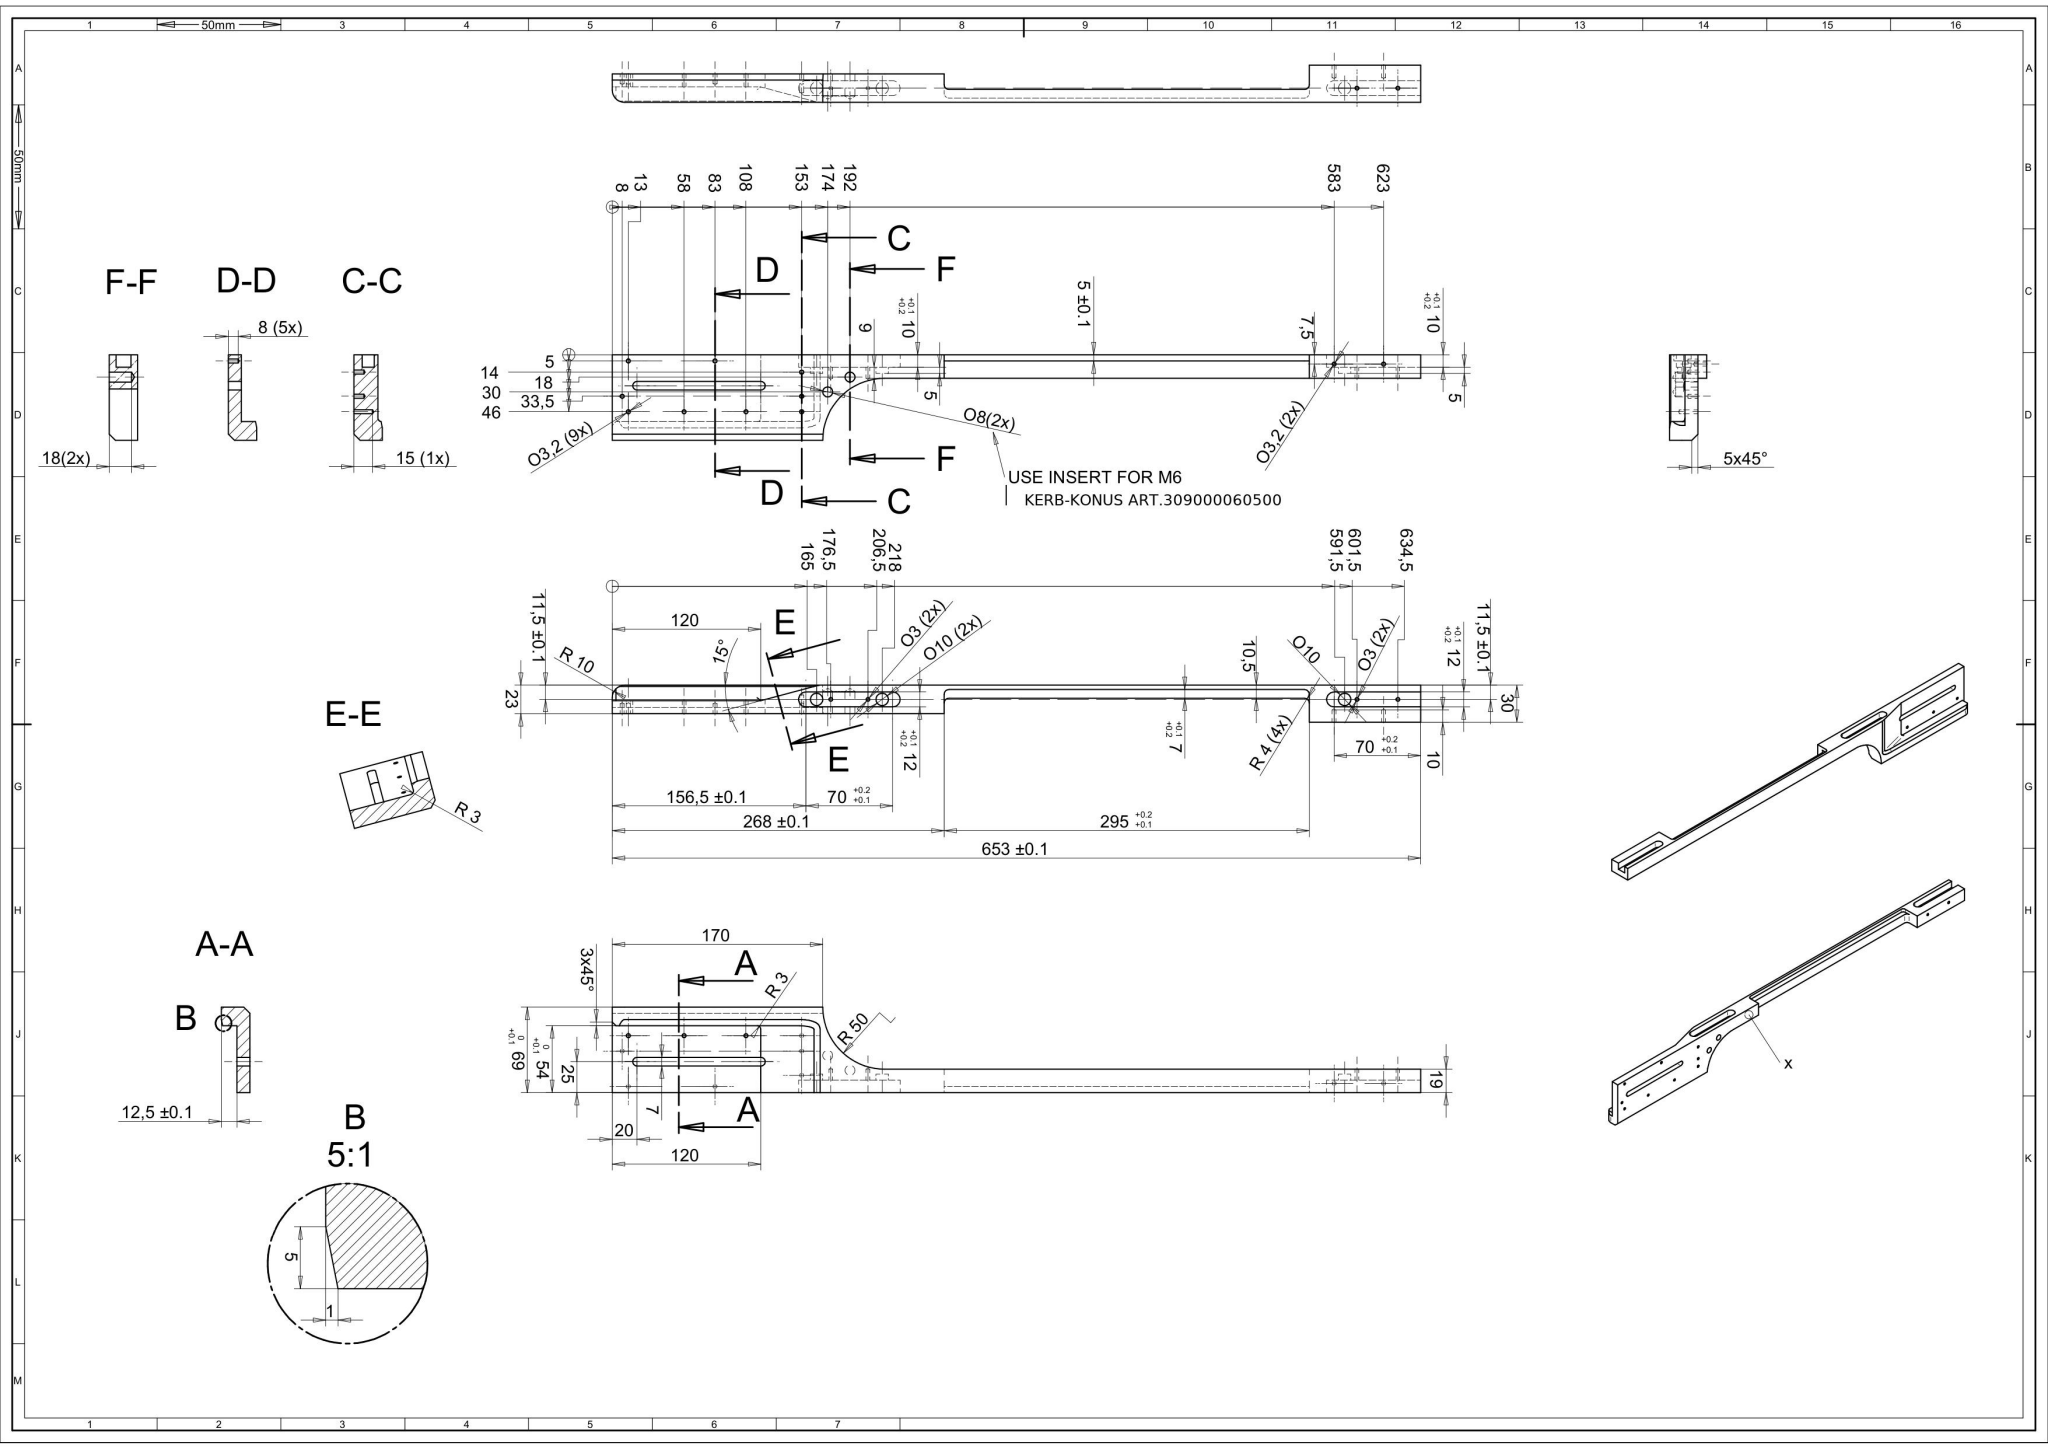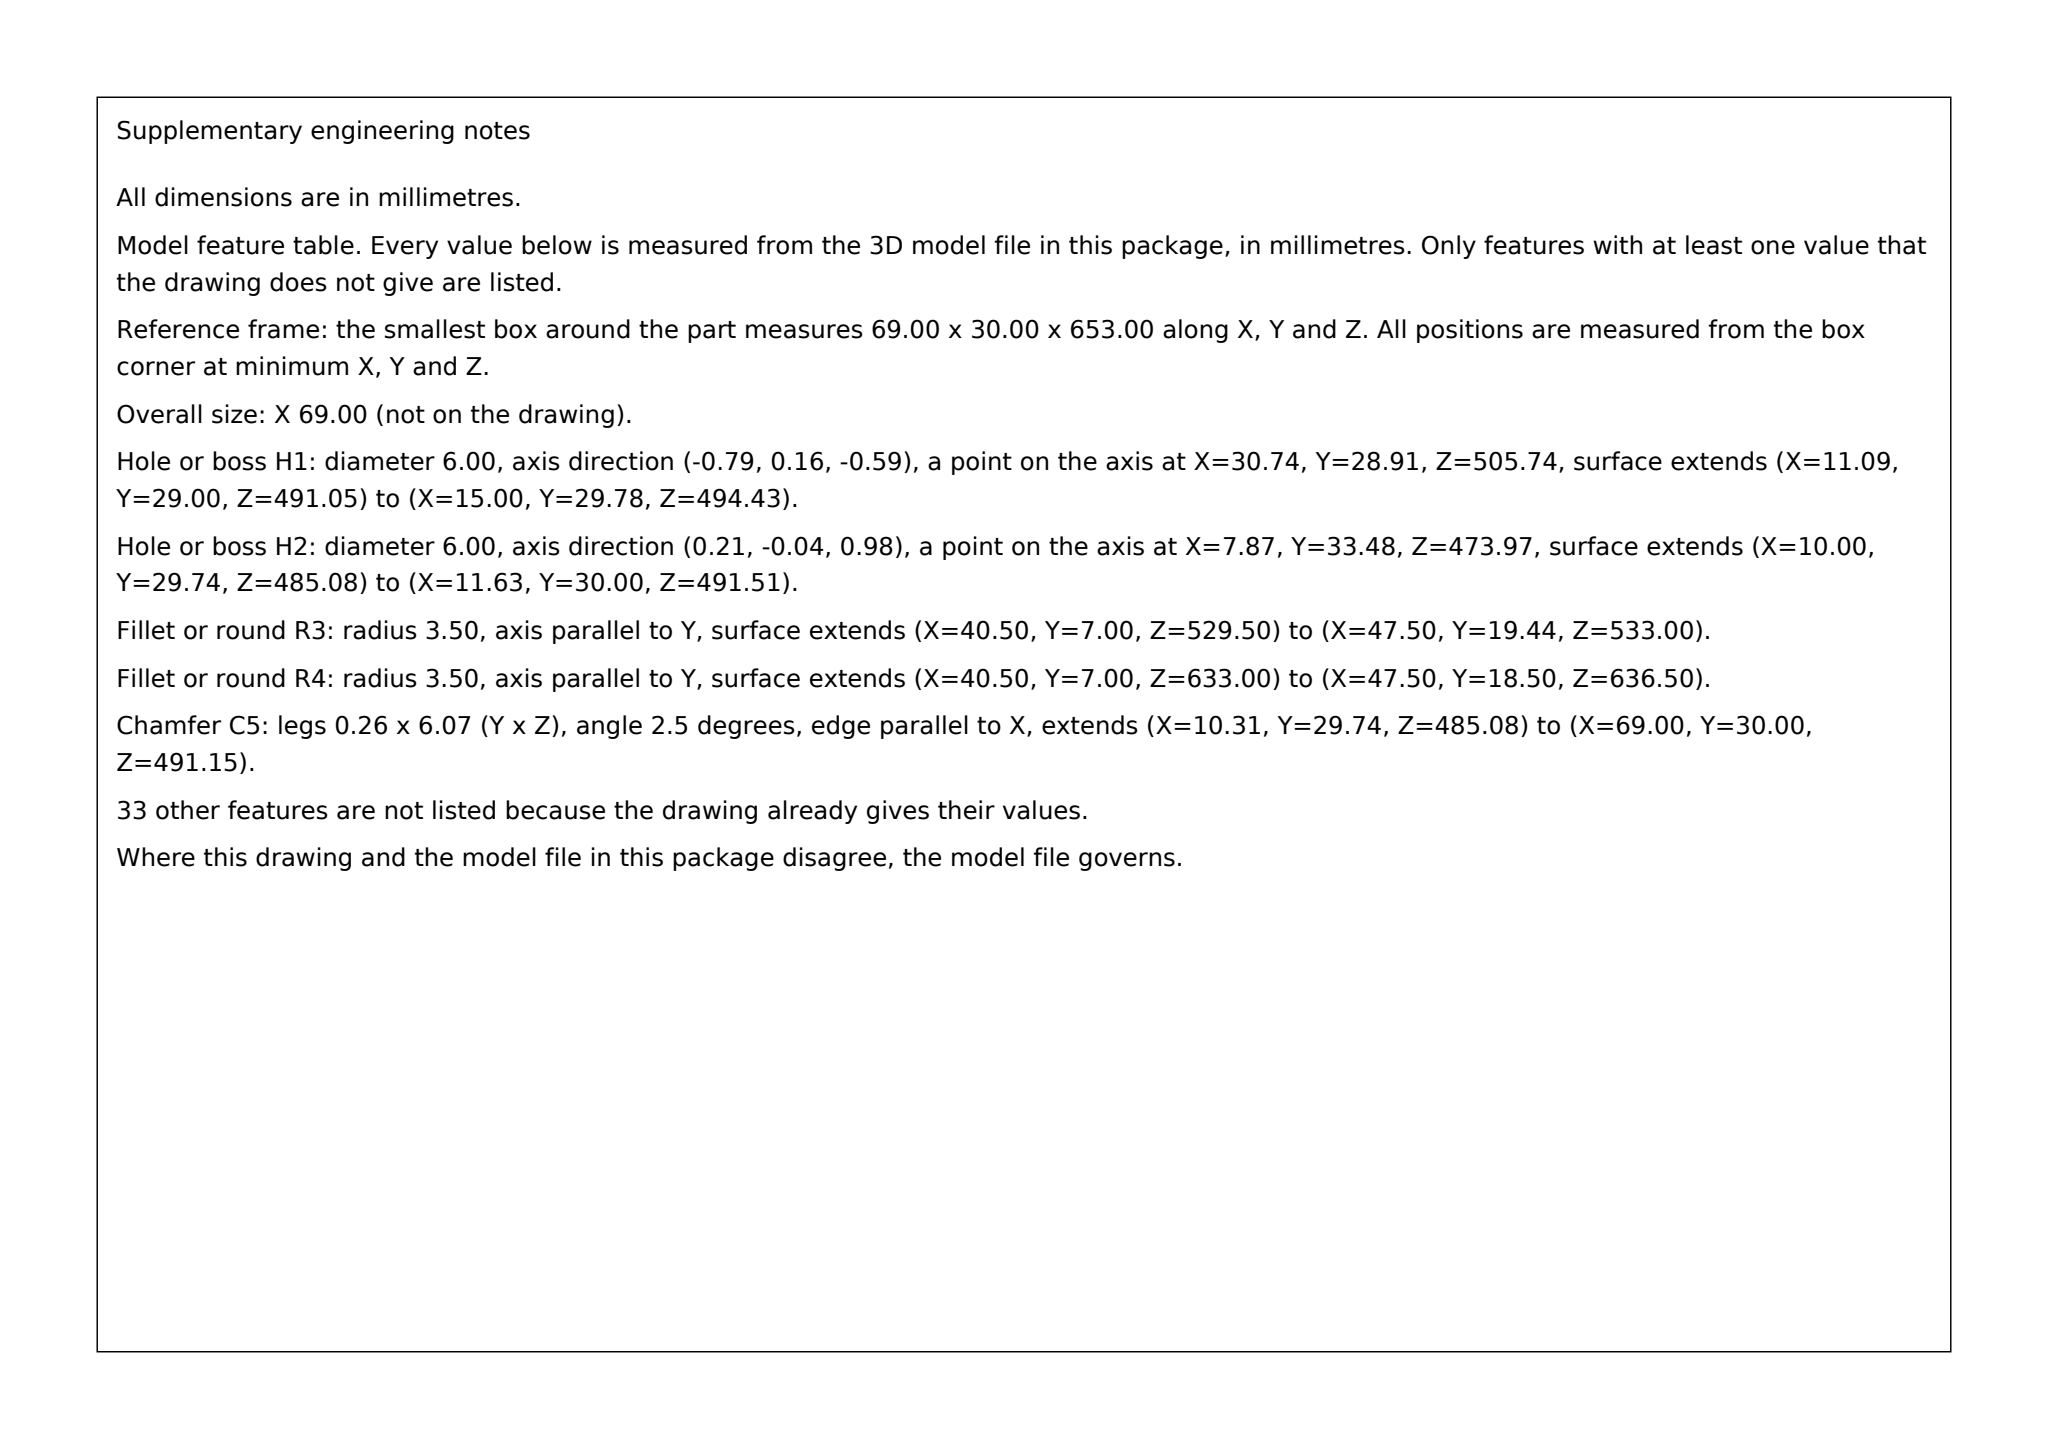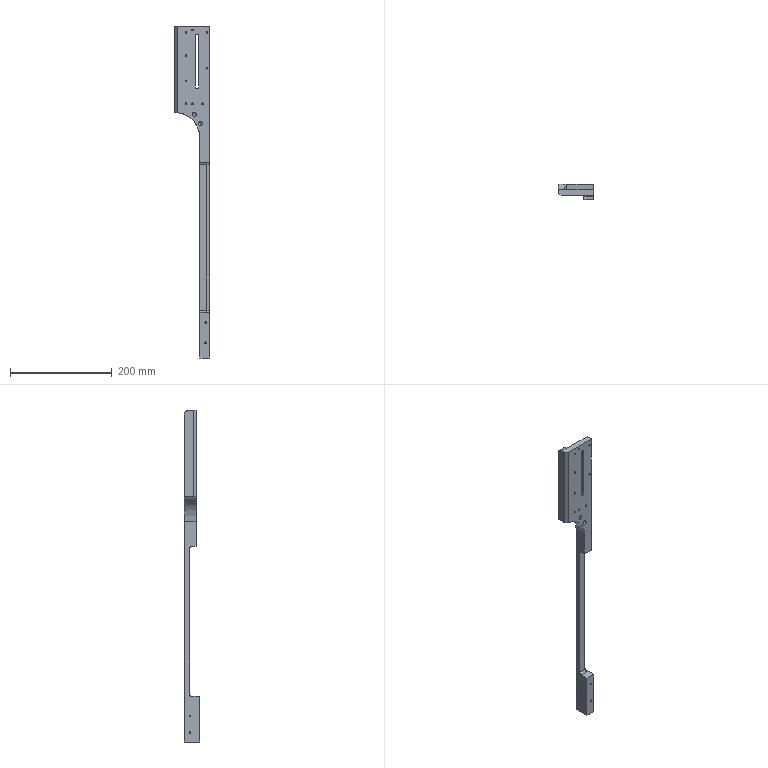Part | SolidWorks | mm | 1 solid | 107 faces | box 69 x 30 x 653 mm | volume 303142 mm3 | cylinder 56 | plane 31 | cone 20 | commonest cylinder face diameters 3.2 x22 8 x8 3 x8 10 x6 12 x4 7 x3 6 x3 100 x1